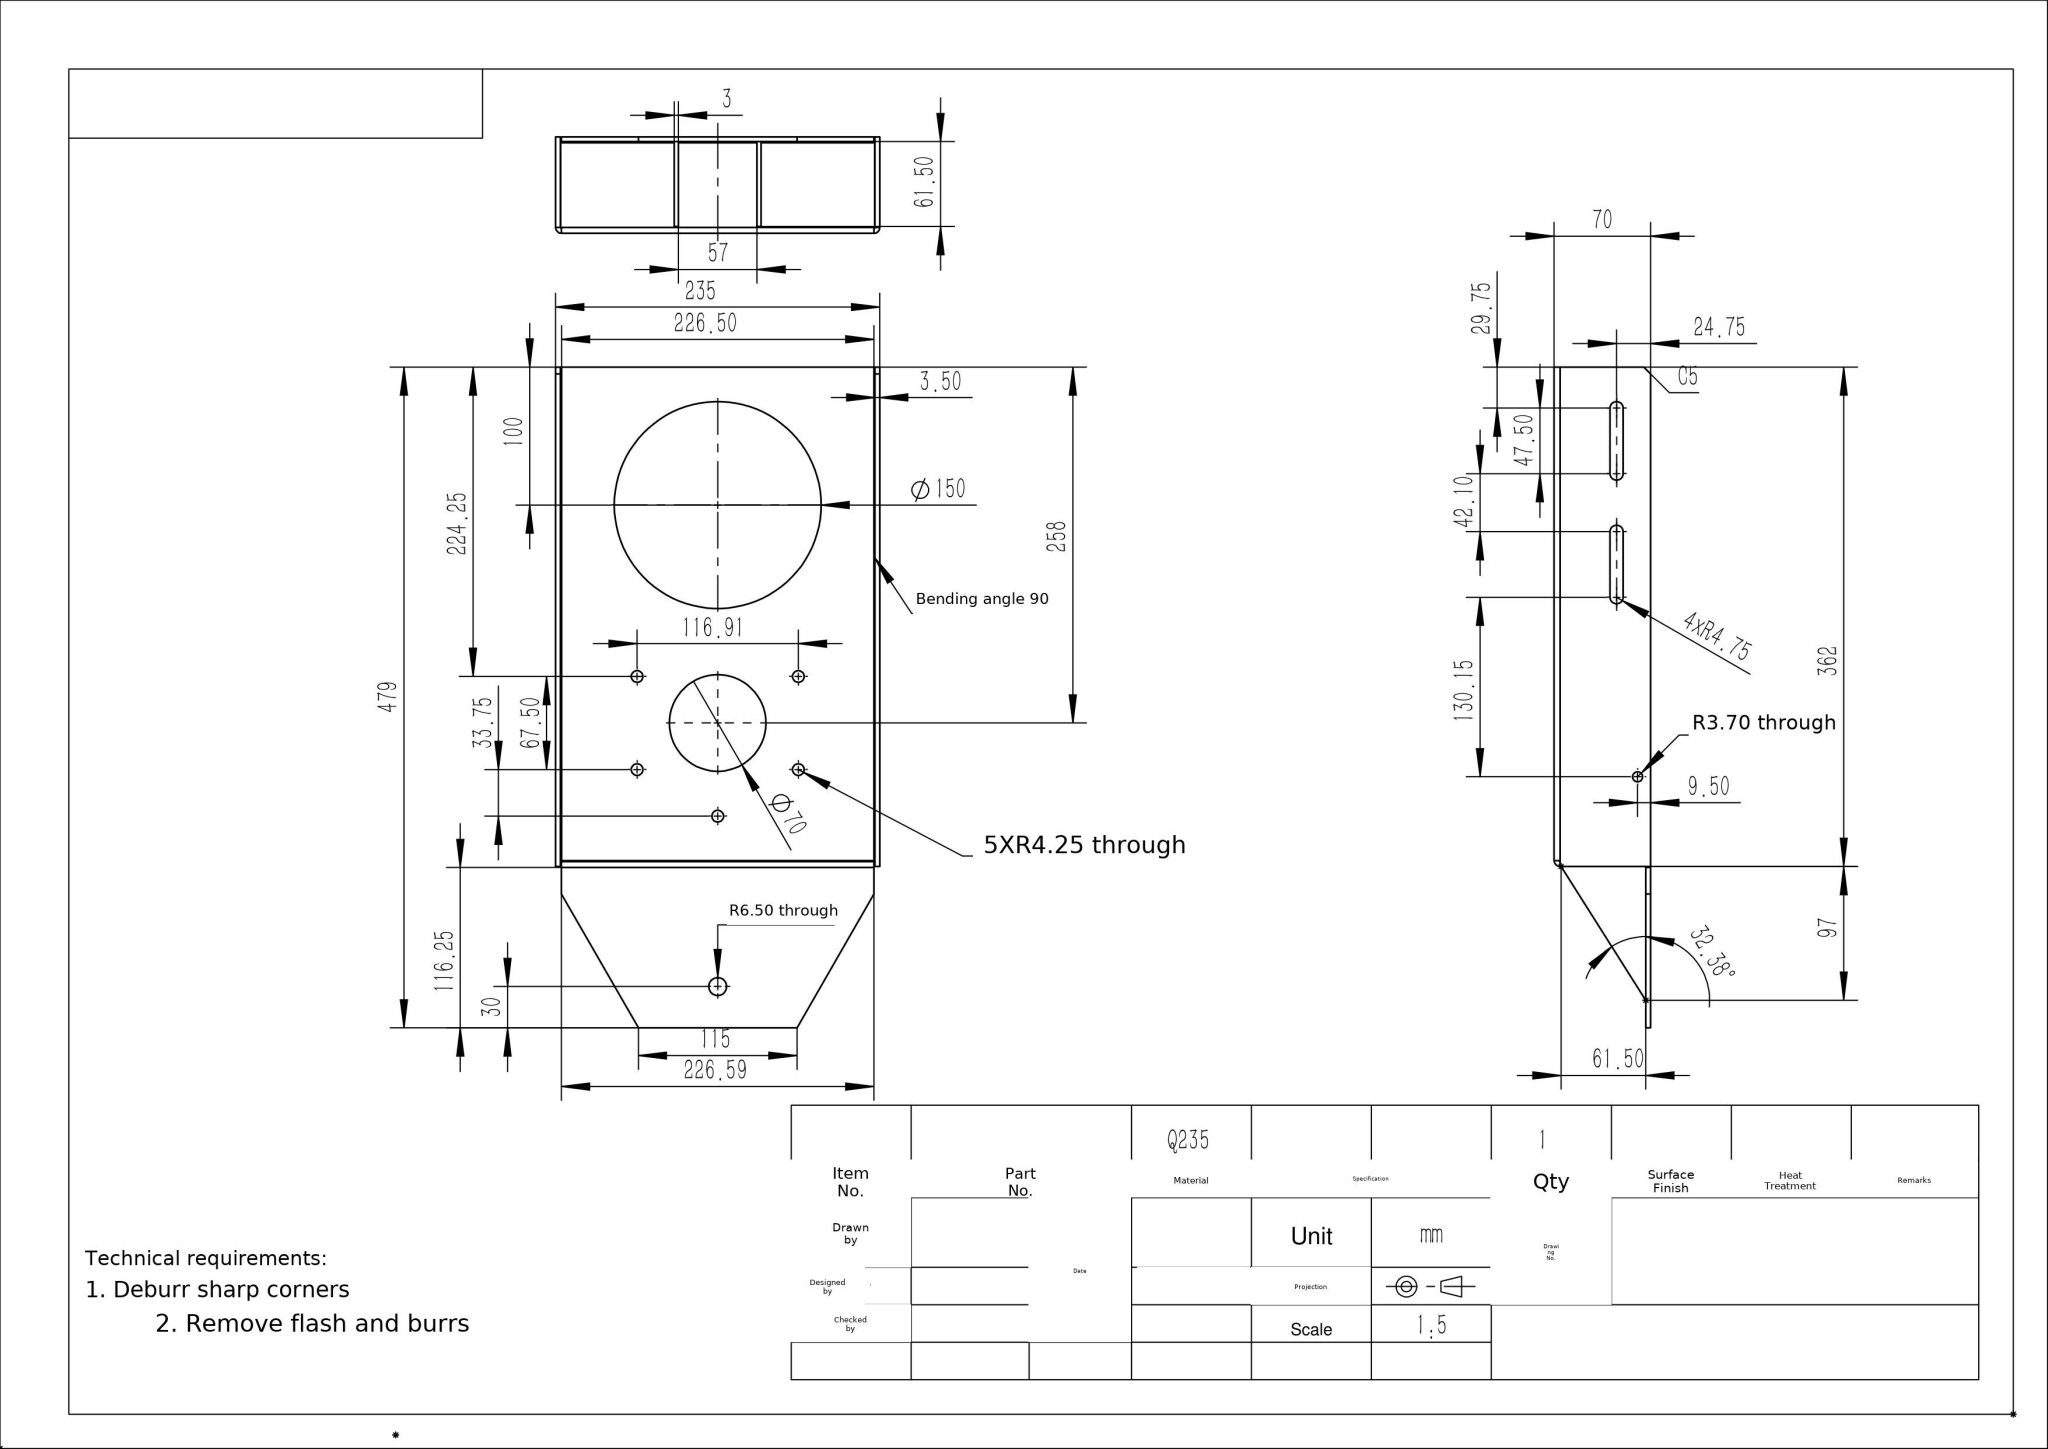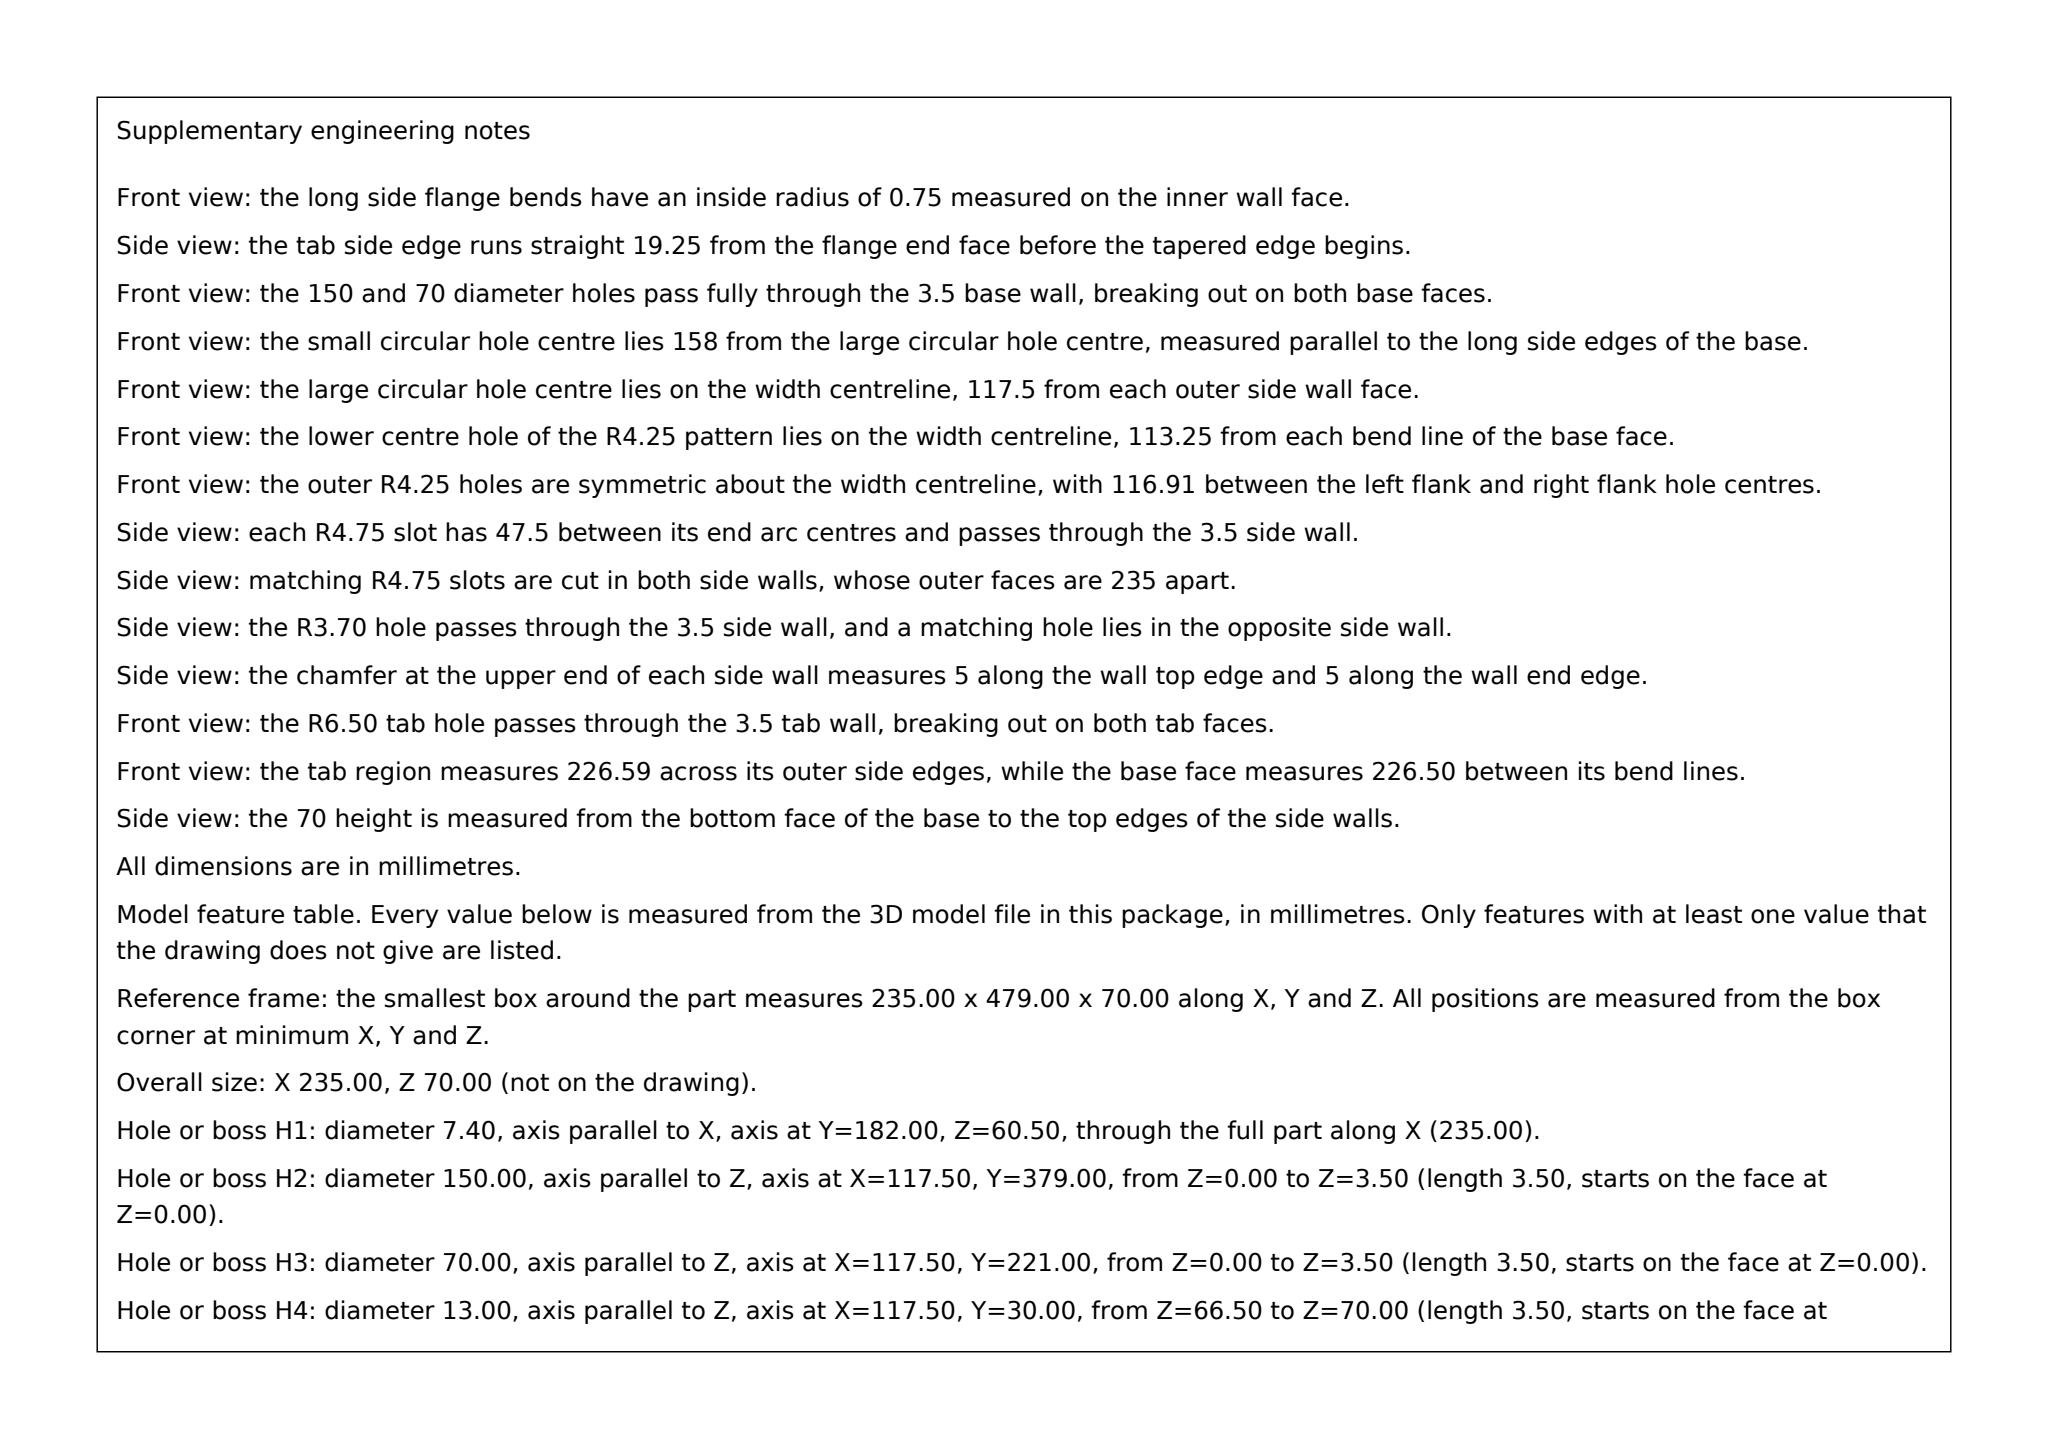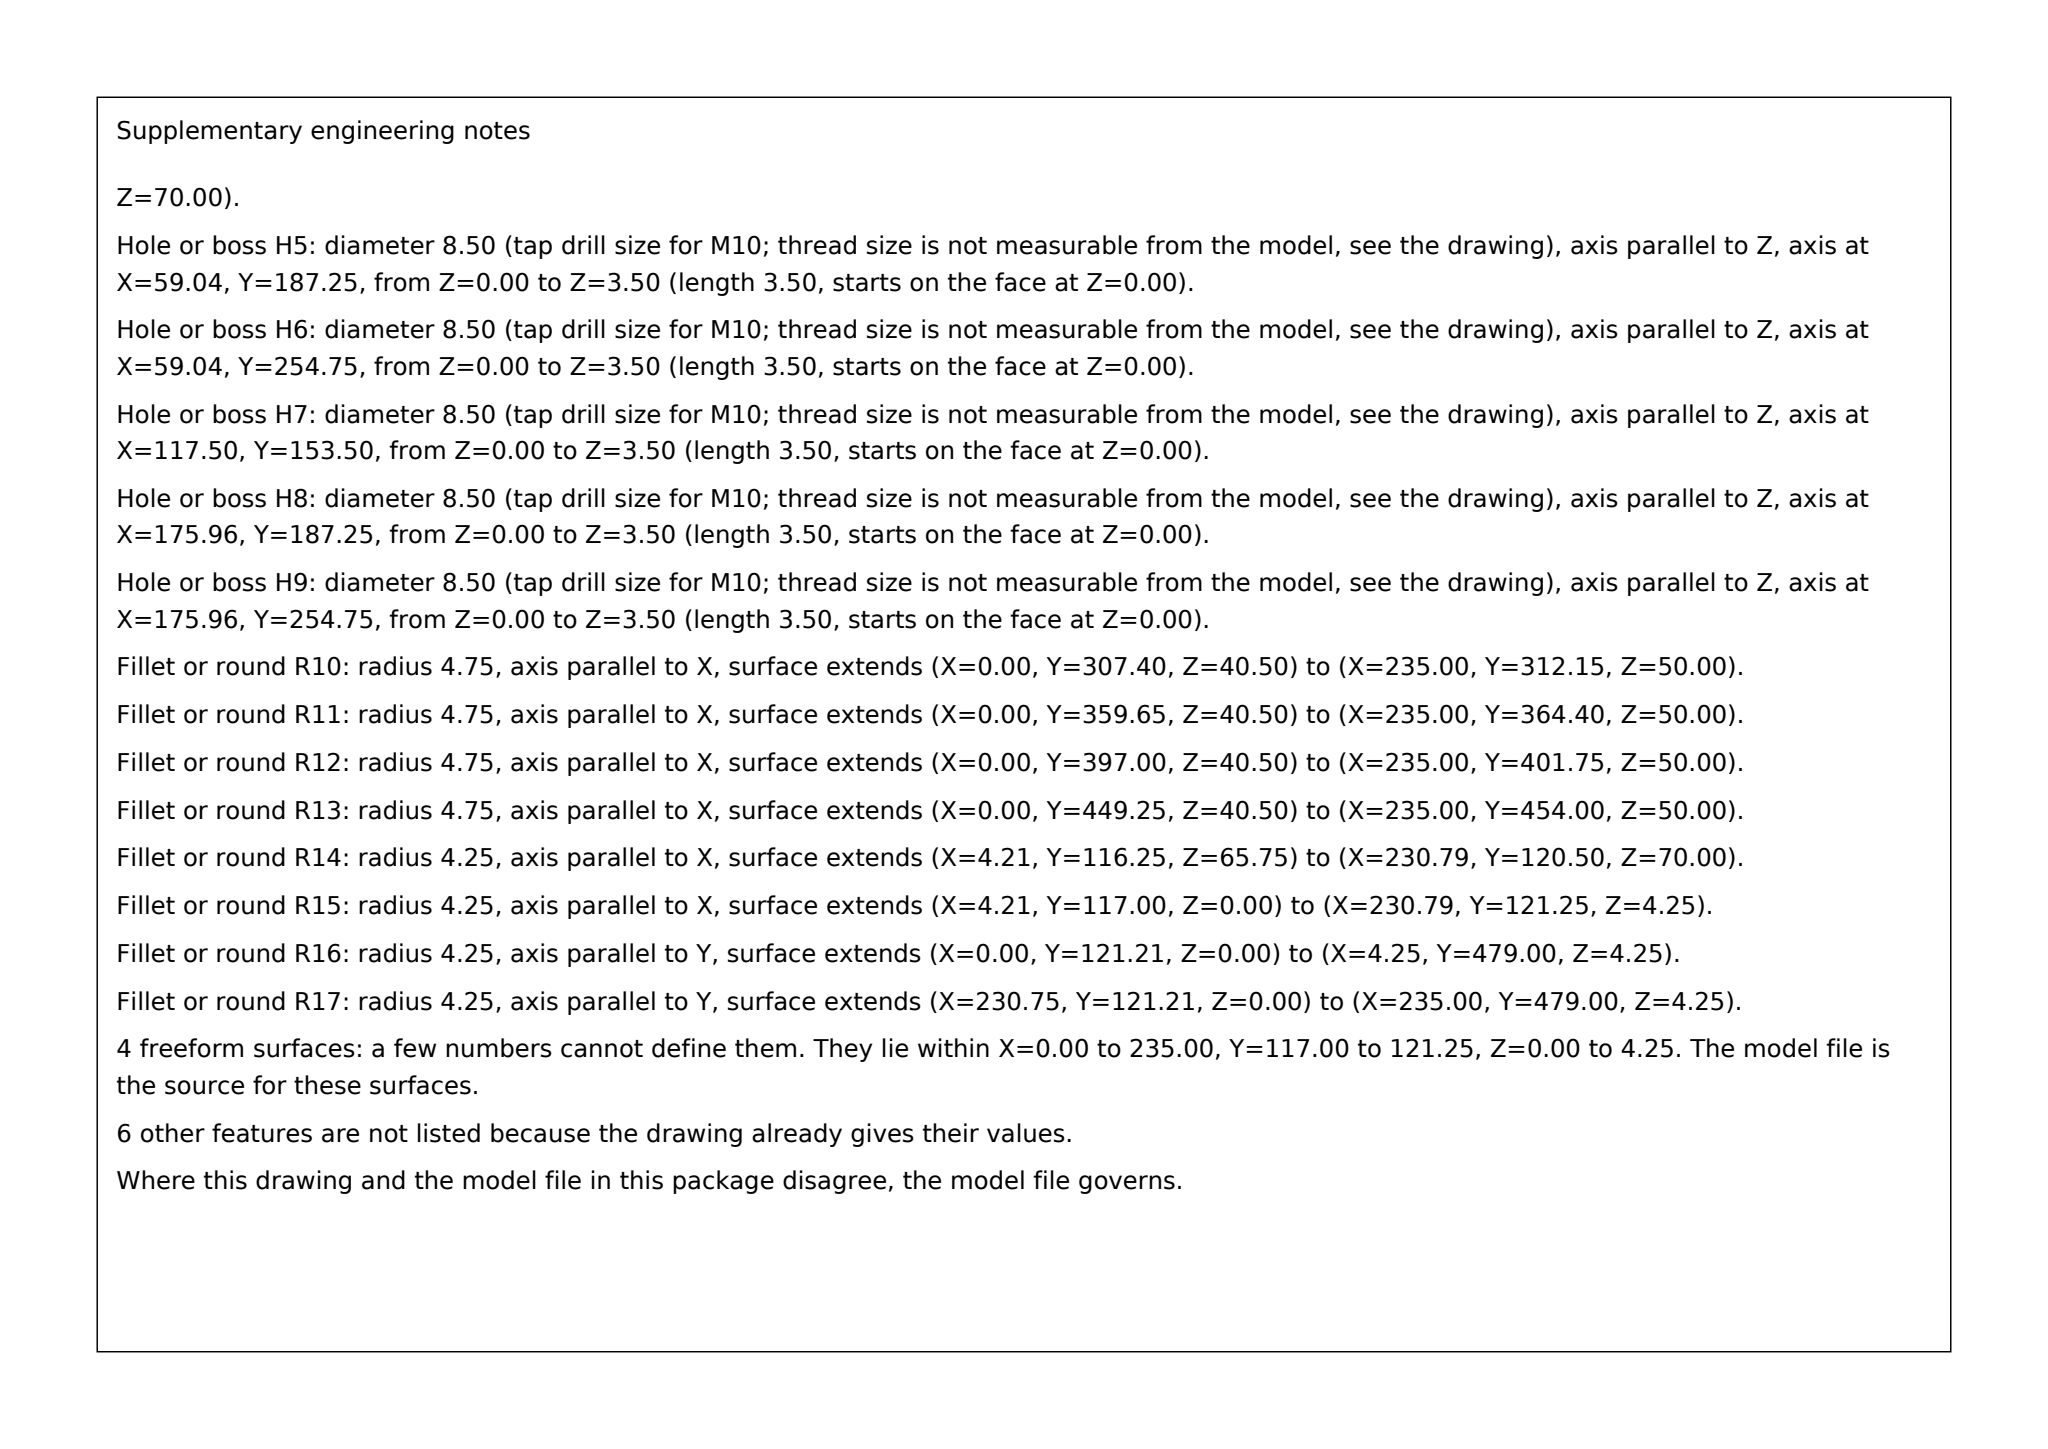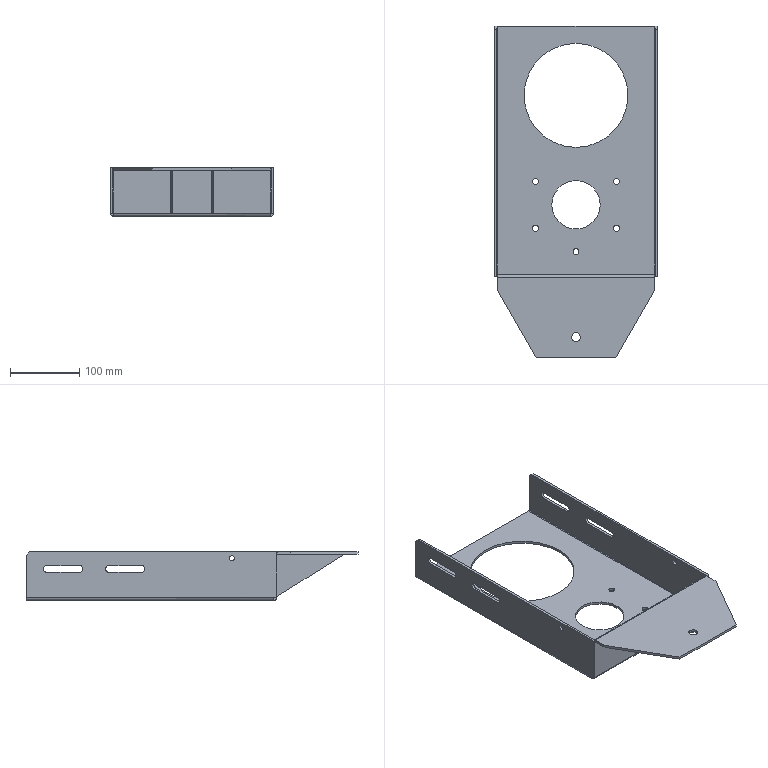Part | SolidWorks | mm | 1 solid | 92 faces | box 235 x 479 x 70 mm | volume 521984 mm3 | plane 50 | cylinder 38 | spline 4 | commonest cylinder face diameters 8.5 x14 9.5 x8 1.5 x6 7.4 x4 70 x2 150 x2 13 x2
Drawing notes:
ALL 90° BENDS: INSIDE BEND R0.75, OUTSIDE R4.25, THK 3.5 | from the solid: Coaxial bend cyls dia 1.5 (R0.75 inner) + dia 8.5 (R4.25 outer) at y-axis x=4.29 & x=230.79 (len 357.79) and x-axis y=121.25 z=4.29 (len 226.59); sheet thk = planes z0.04/z3.54 = 3.5
32.38° BEND: INSIDE R0.75, OUTSIDE R4.25, THK 3.5 | from the solid: Coaxial cyls dia 1.5 & dia 8.5 on x-axis at y=116.25, z=65.79 (len 57 and 81.79) at lower tab bend; thk 3.5
LOWER 4XR4.75 SLOT: 47.50 BTWN CTRS, 57 OAL | from the solid: Slot end cyls dia 9.5 x-axis at y=312.15 & y=359.65 (z=45.29): 359.65-312.15=47.50 ctrs, +9.5 = 57.00 end-to-end; 479-359.65=119.35 from top edge matches 29.75+47.50+42.10